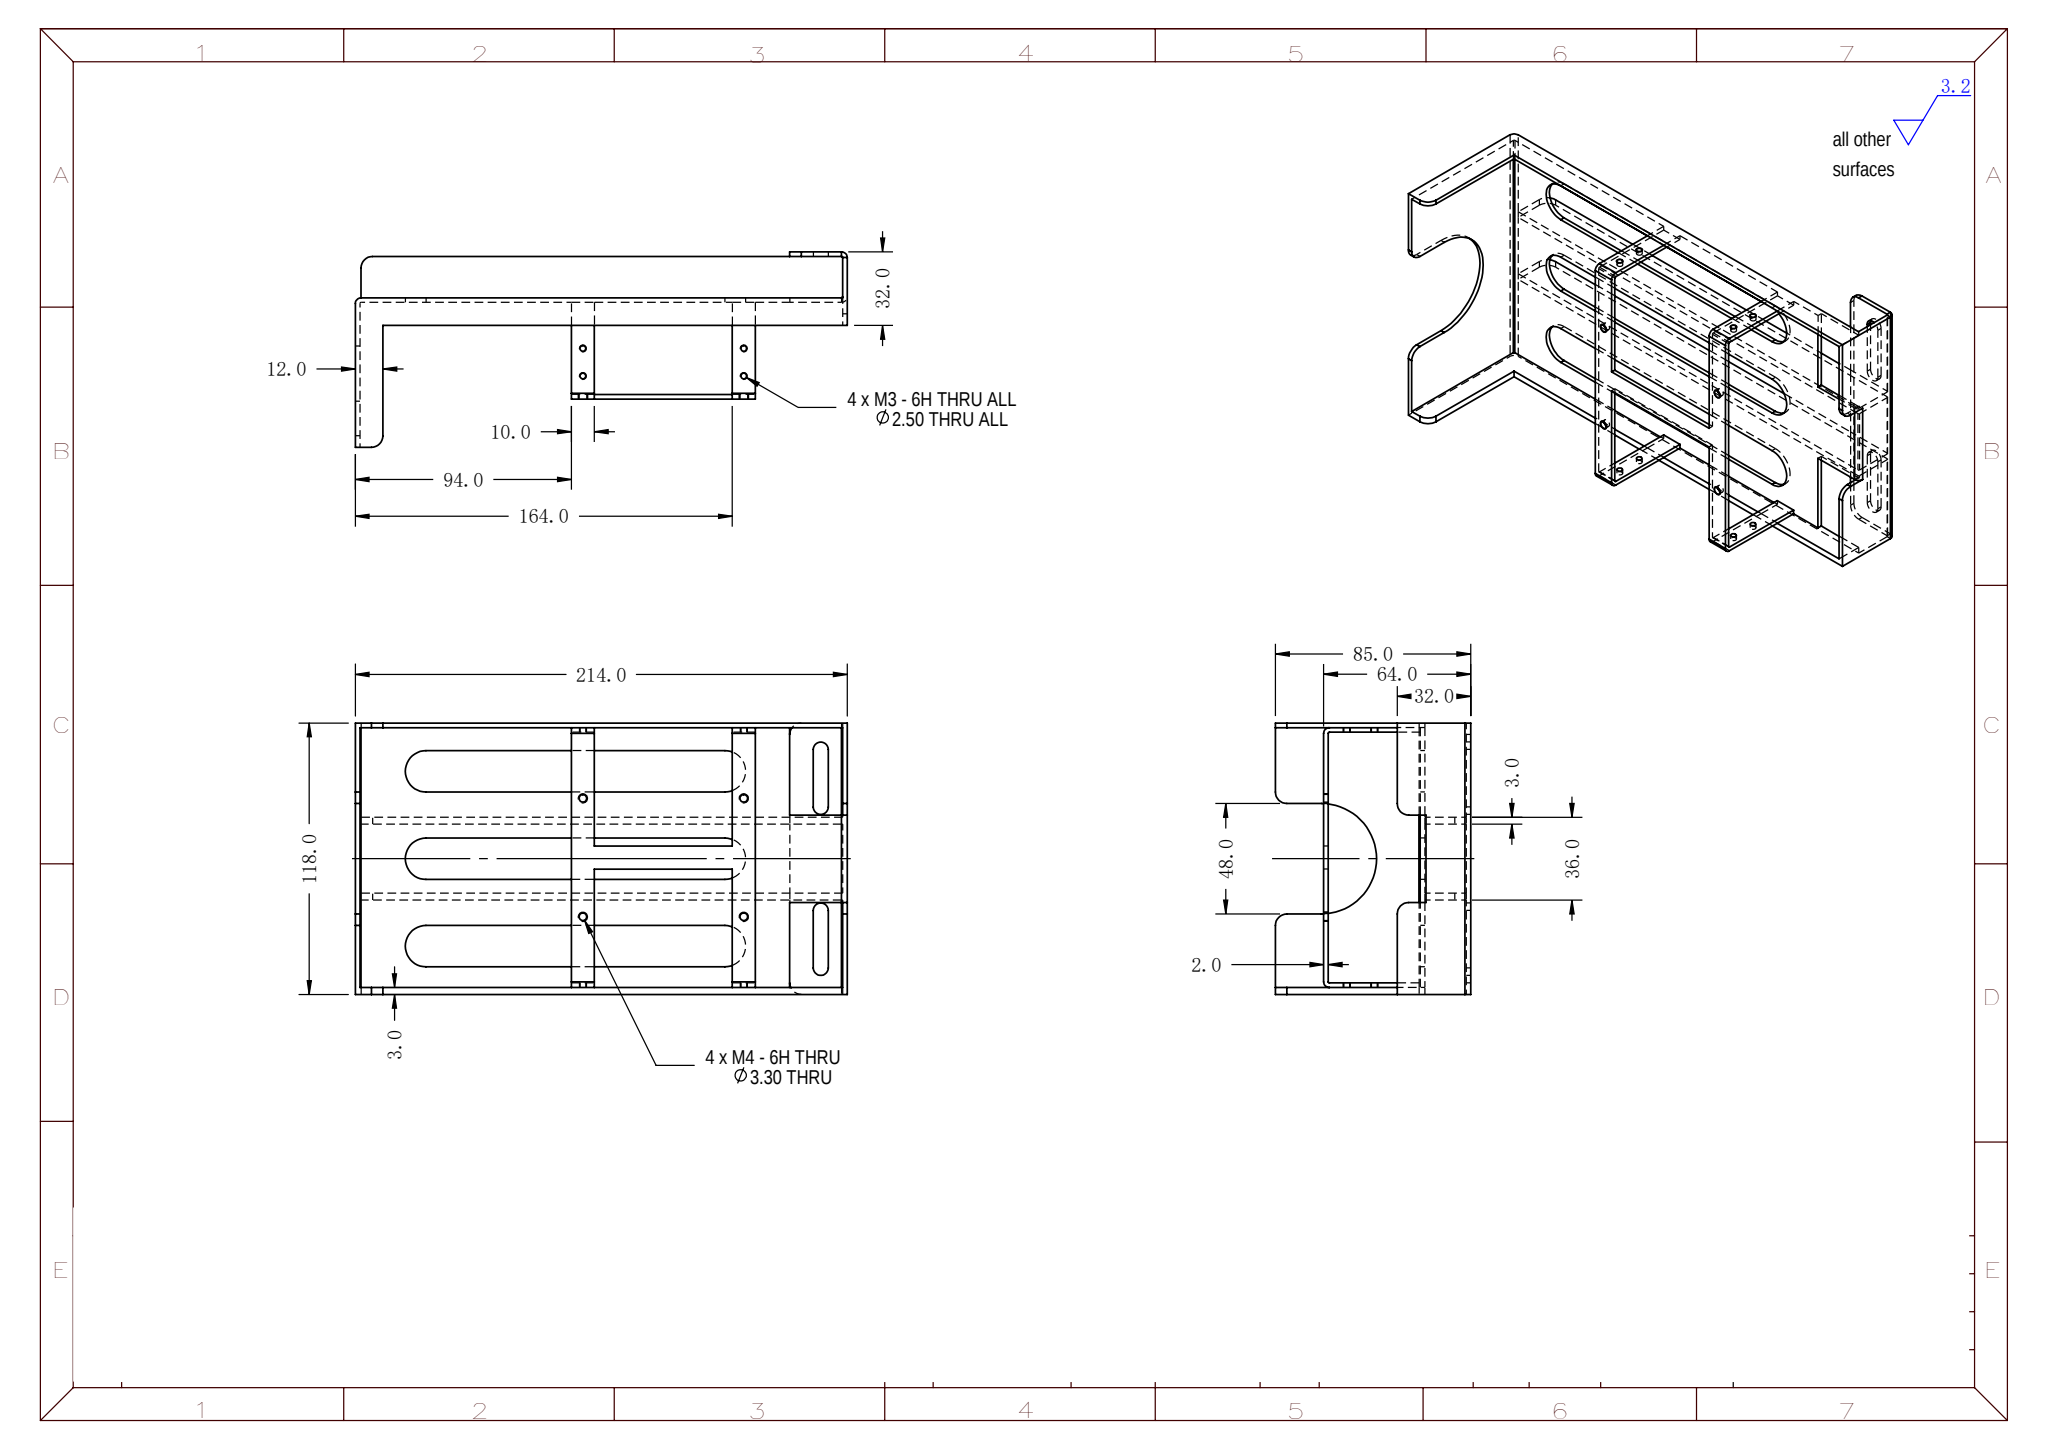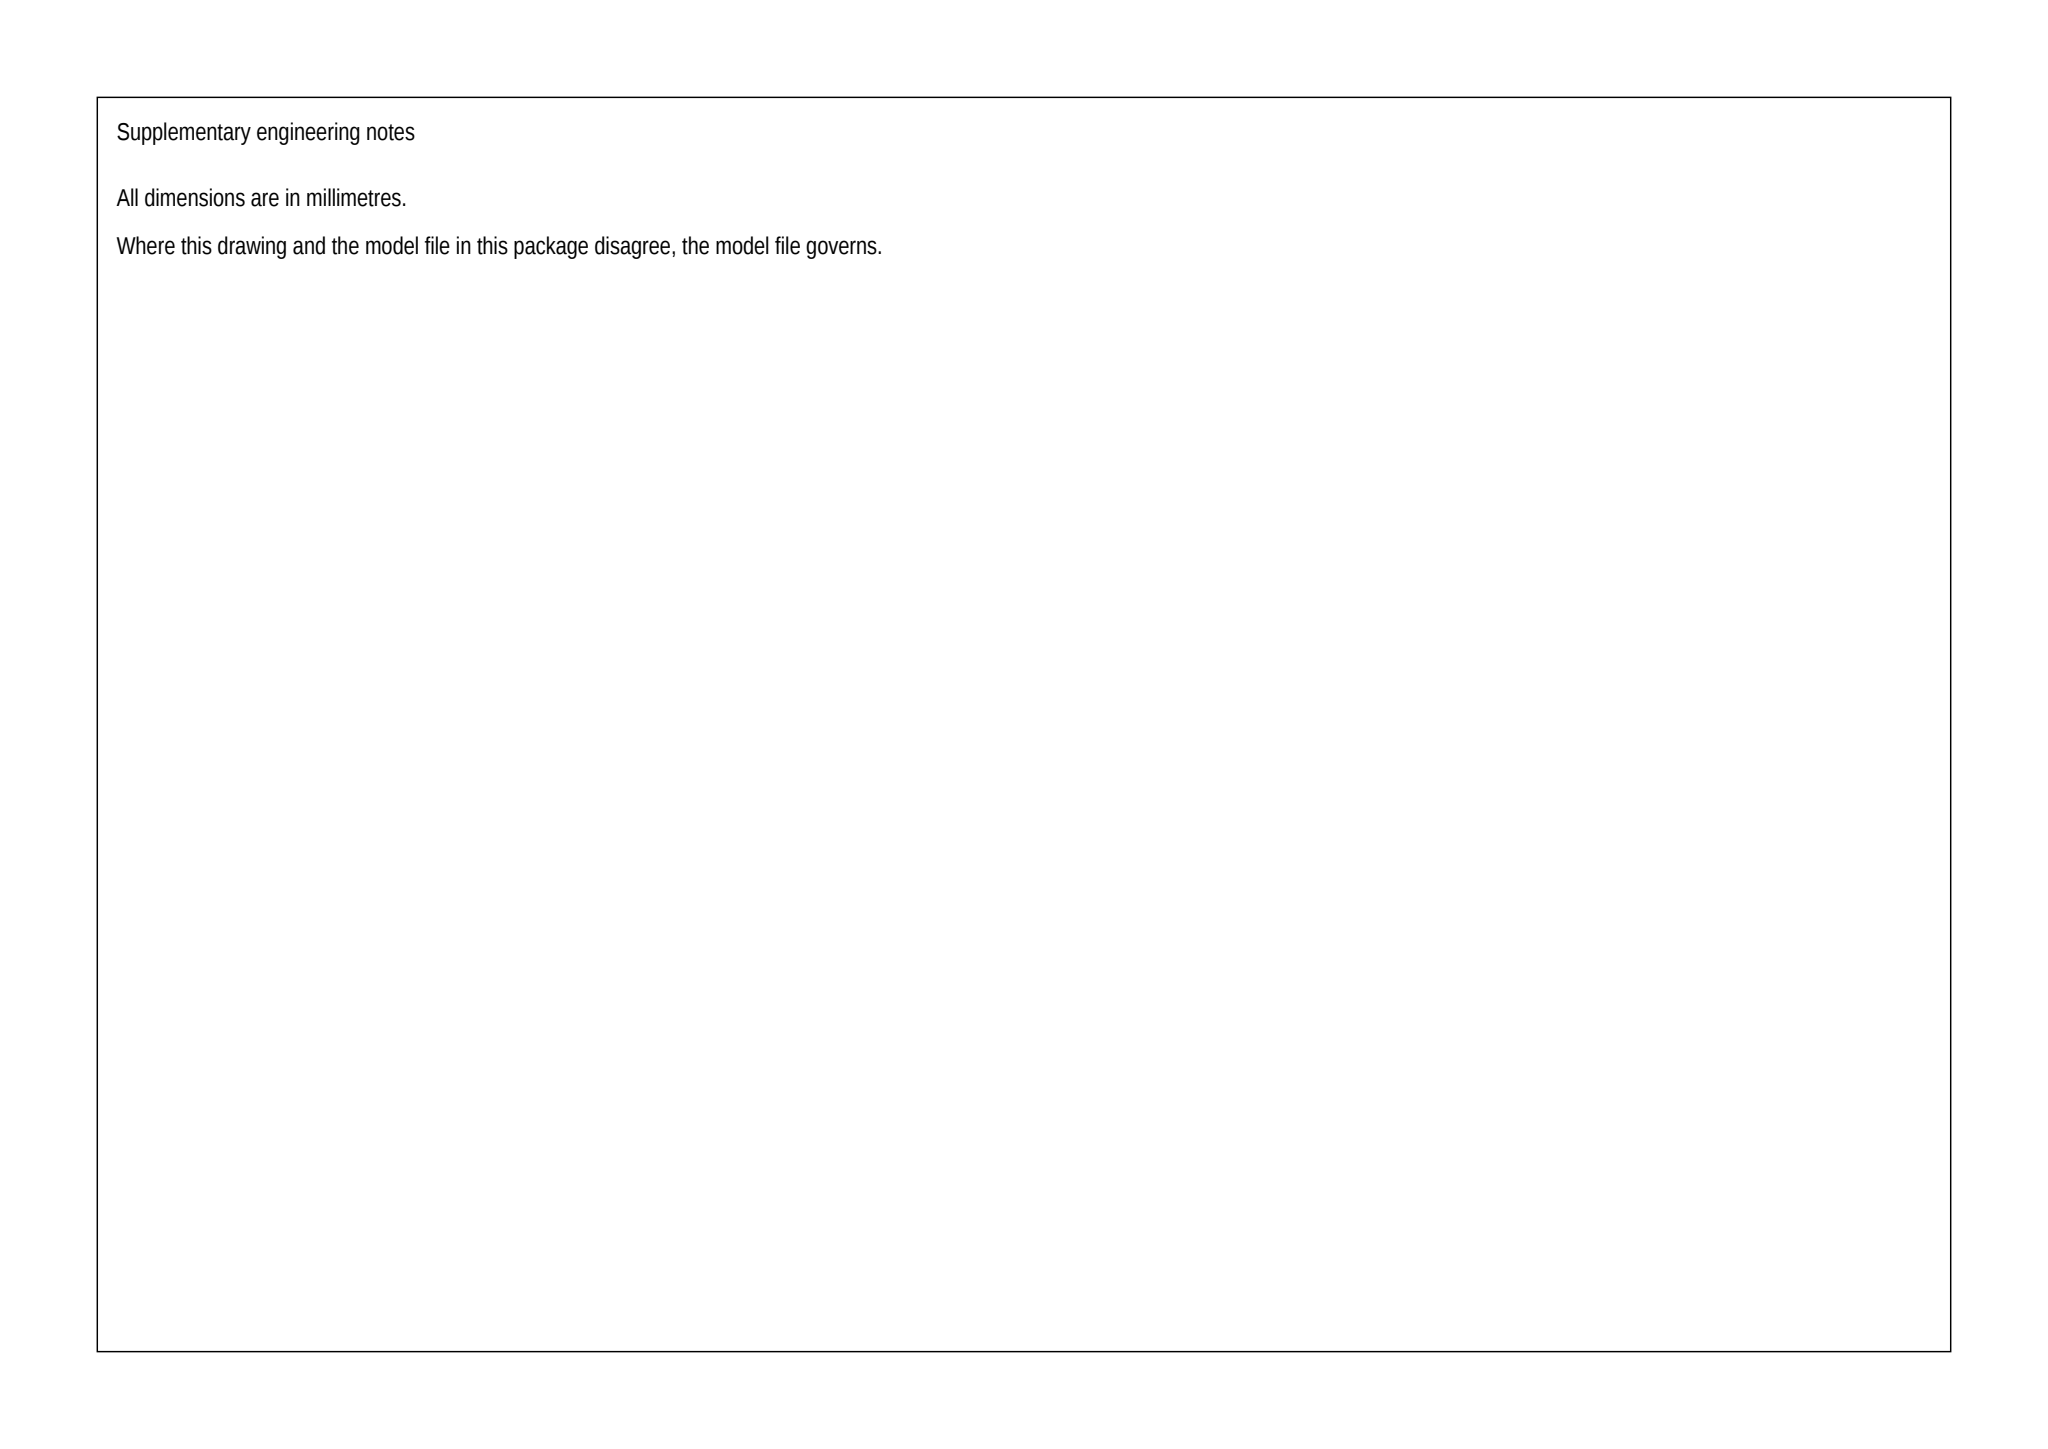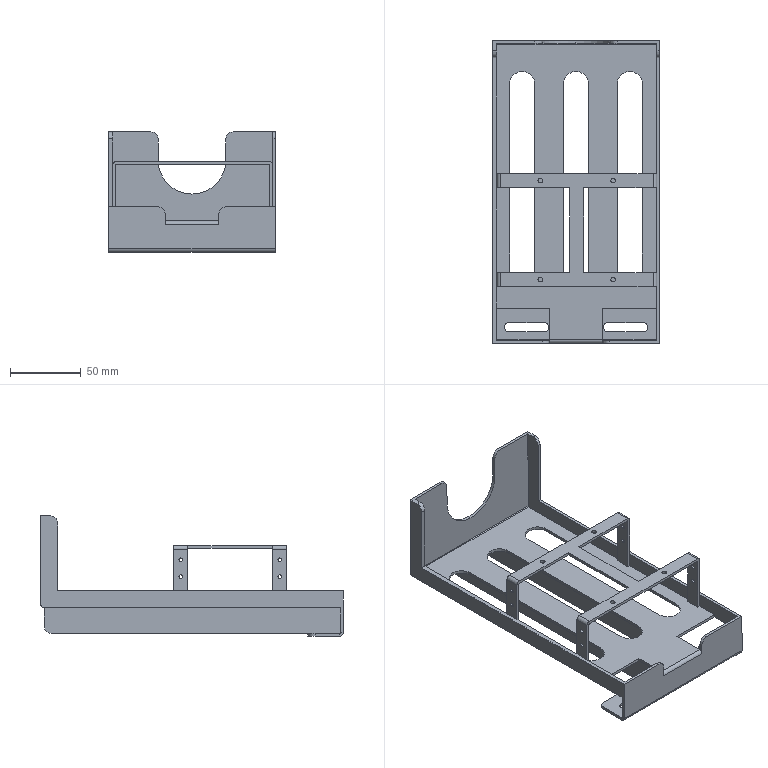Part | SolidWorks | mm | 1 solid | 145 faces | box 118 x 214 x 85 mm | volume 97611 mm3 | plane 79 | cylinder 66 | commonest cylinder face diameters 2.5 x16 1 x11 10 x10 3.3 x8 5 x7 6.5 x6 18 x6 48 x2